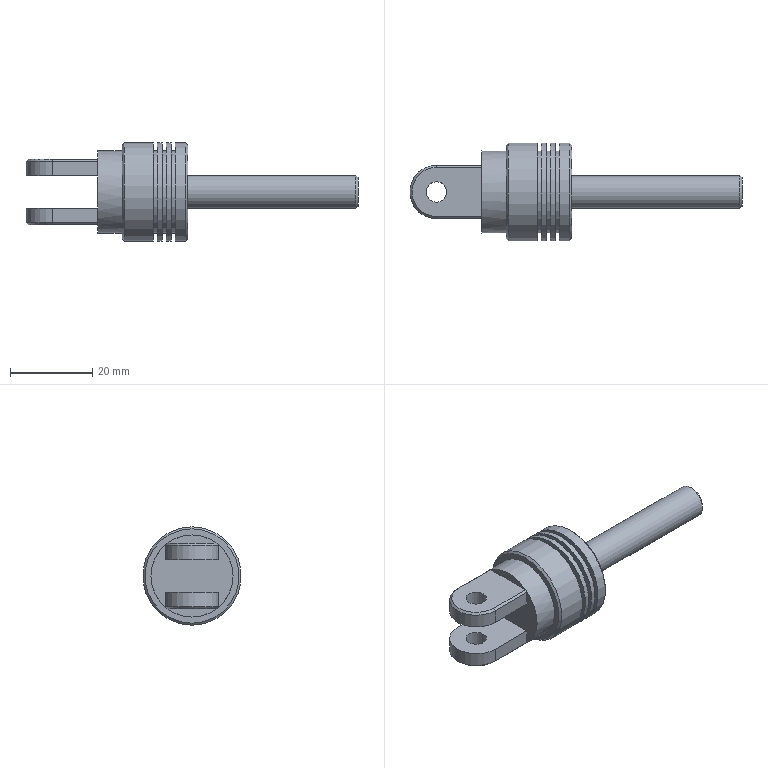Component | NX | PISTON | 1 solid | 42 faces | volume 12280 mm3 | plane 24 | cylinder 13 | cone 5 | commonest cylinder face diameters 20 x4 24 x4 13 x2 5 x2 8 x1